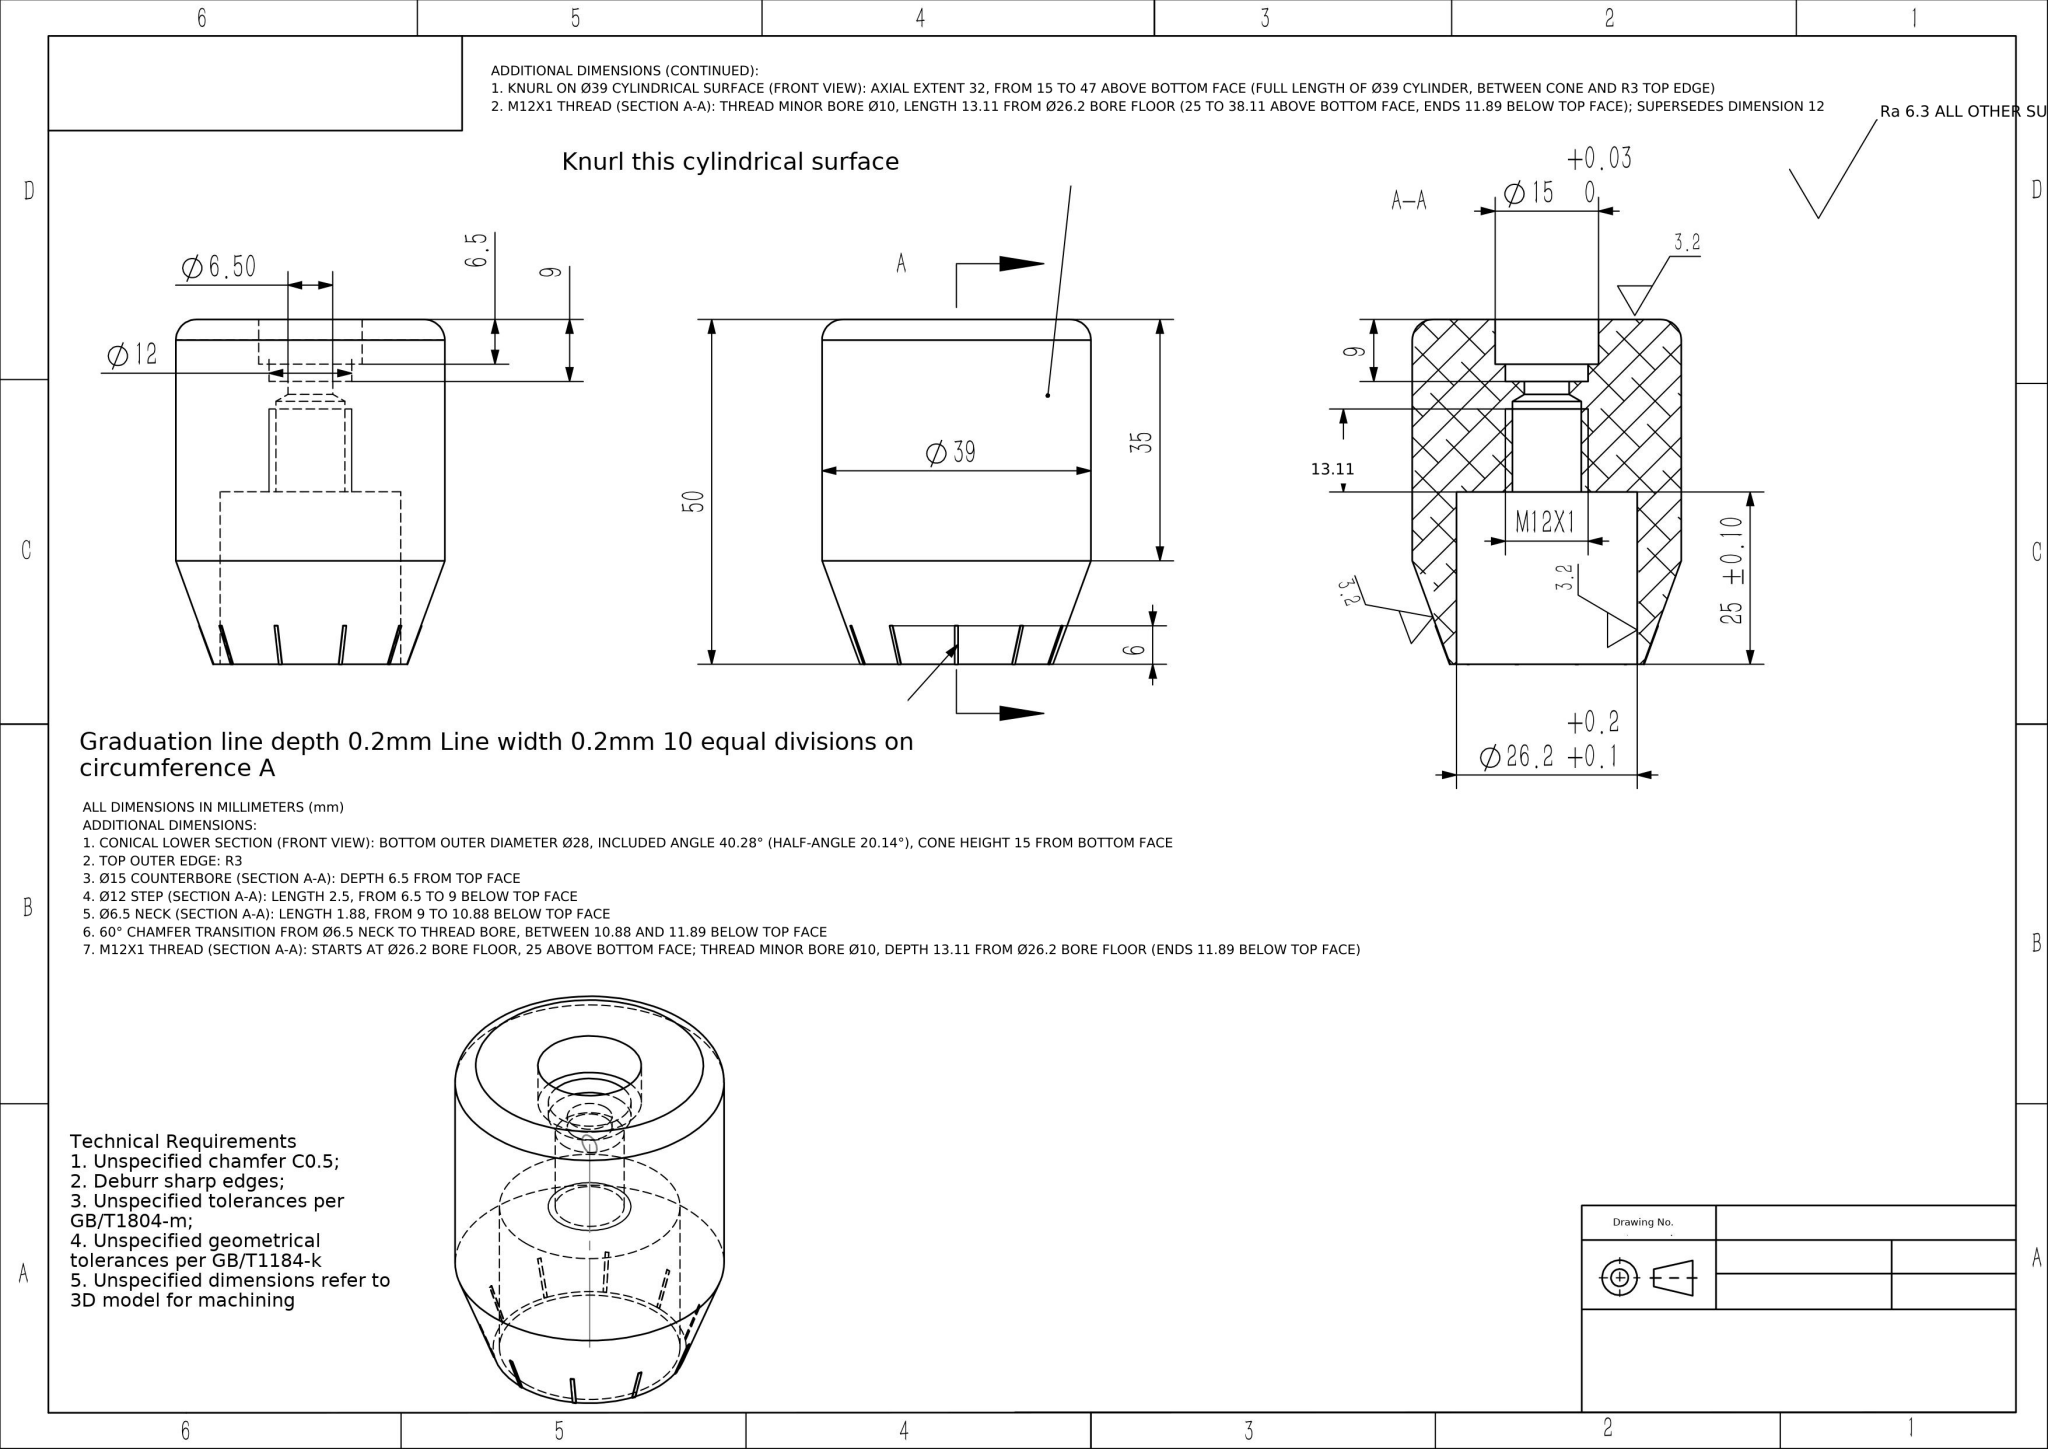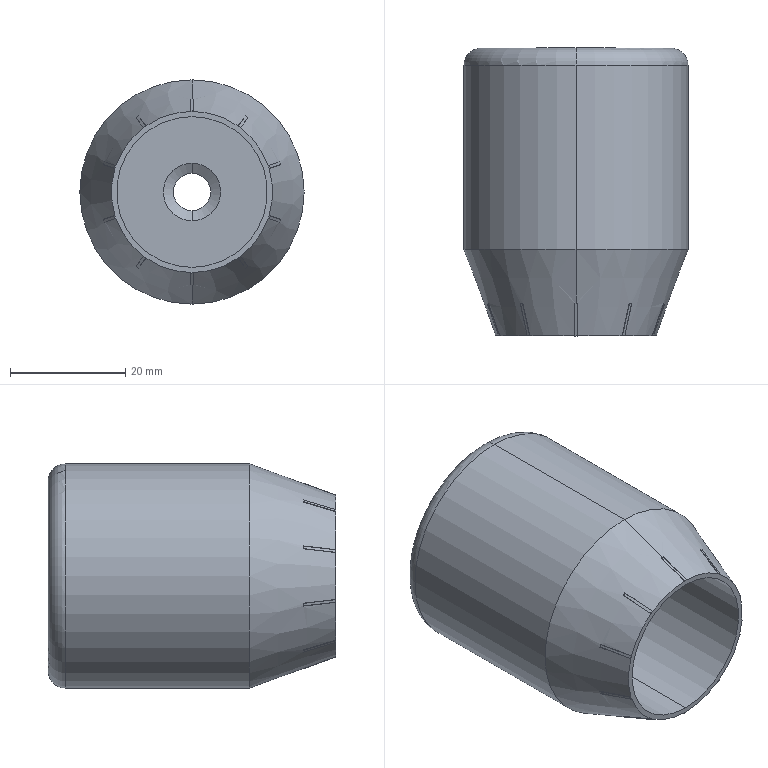Part | NX | mm | 1 solid | 73 faces | box 39 x 50.03 x 39 mm | volume 38868 mm3 | plane 55 | cylinder 12 | cone 4 | torus 2 | commonest cylinder face diameters 12 x2 15 x2 10 x2 39 x2 26.2 x2 6.5 x2